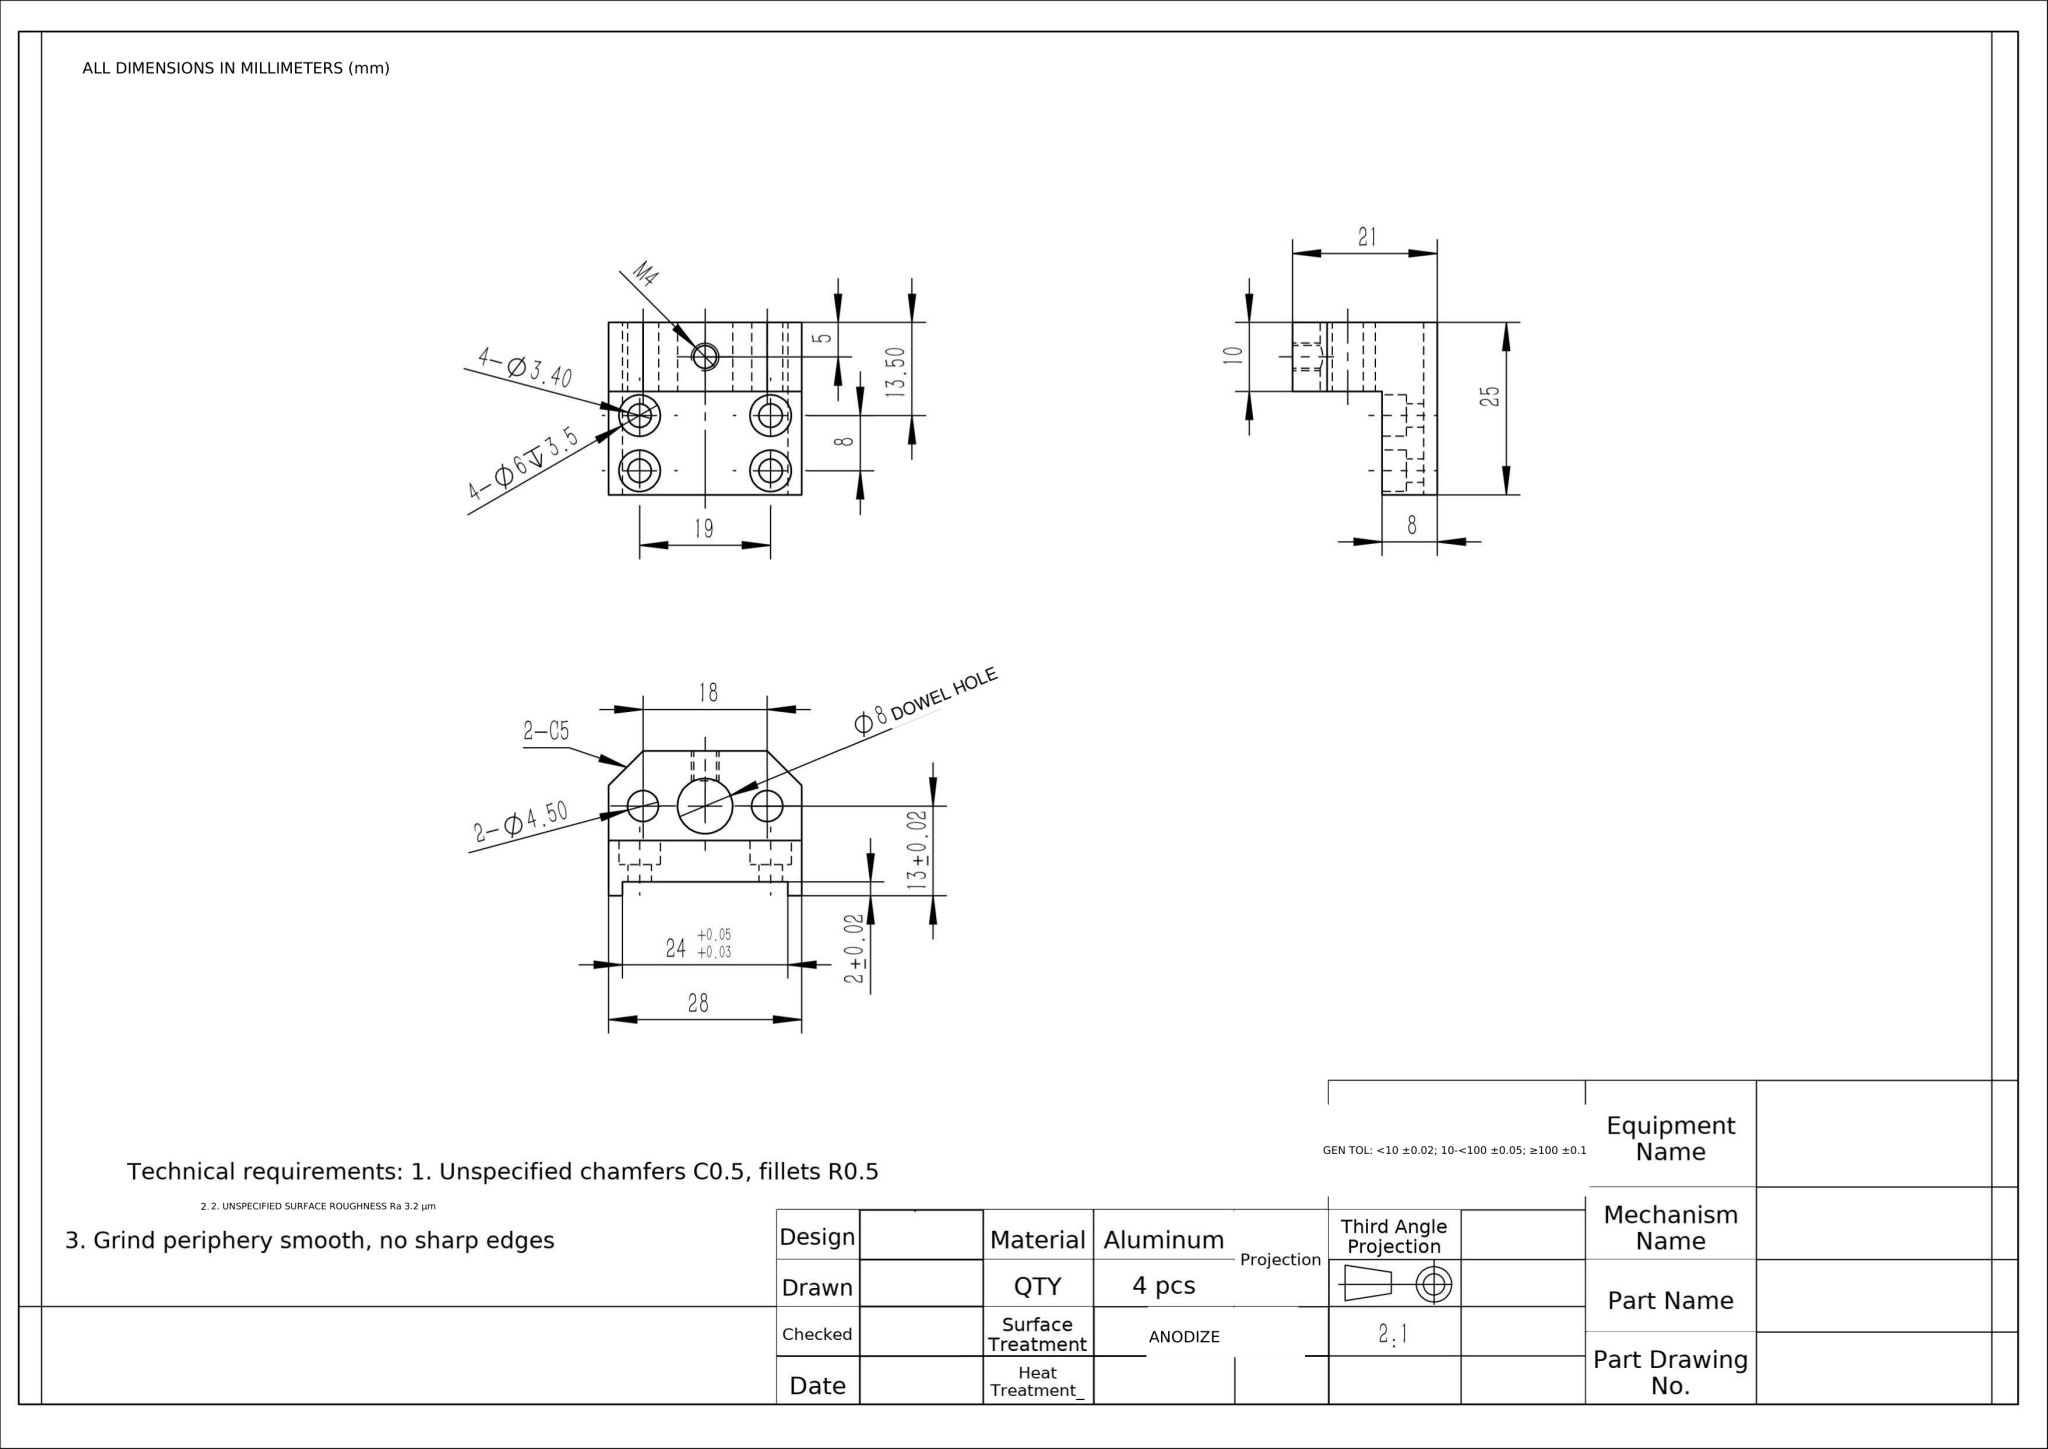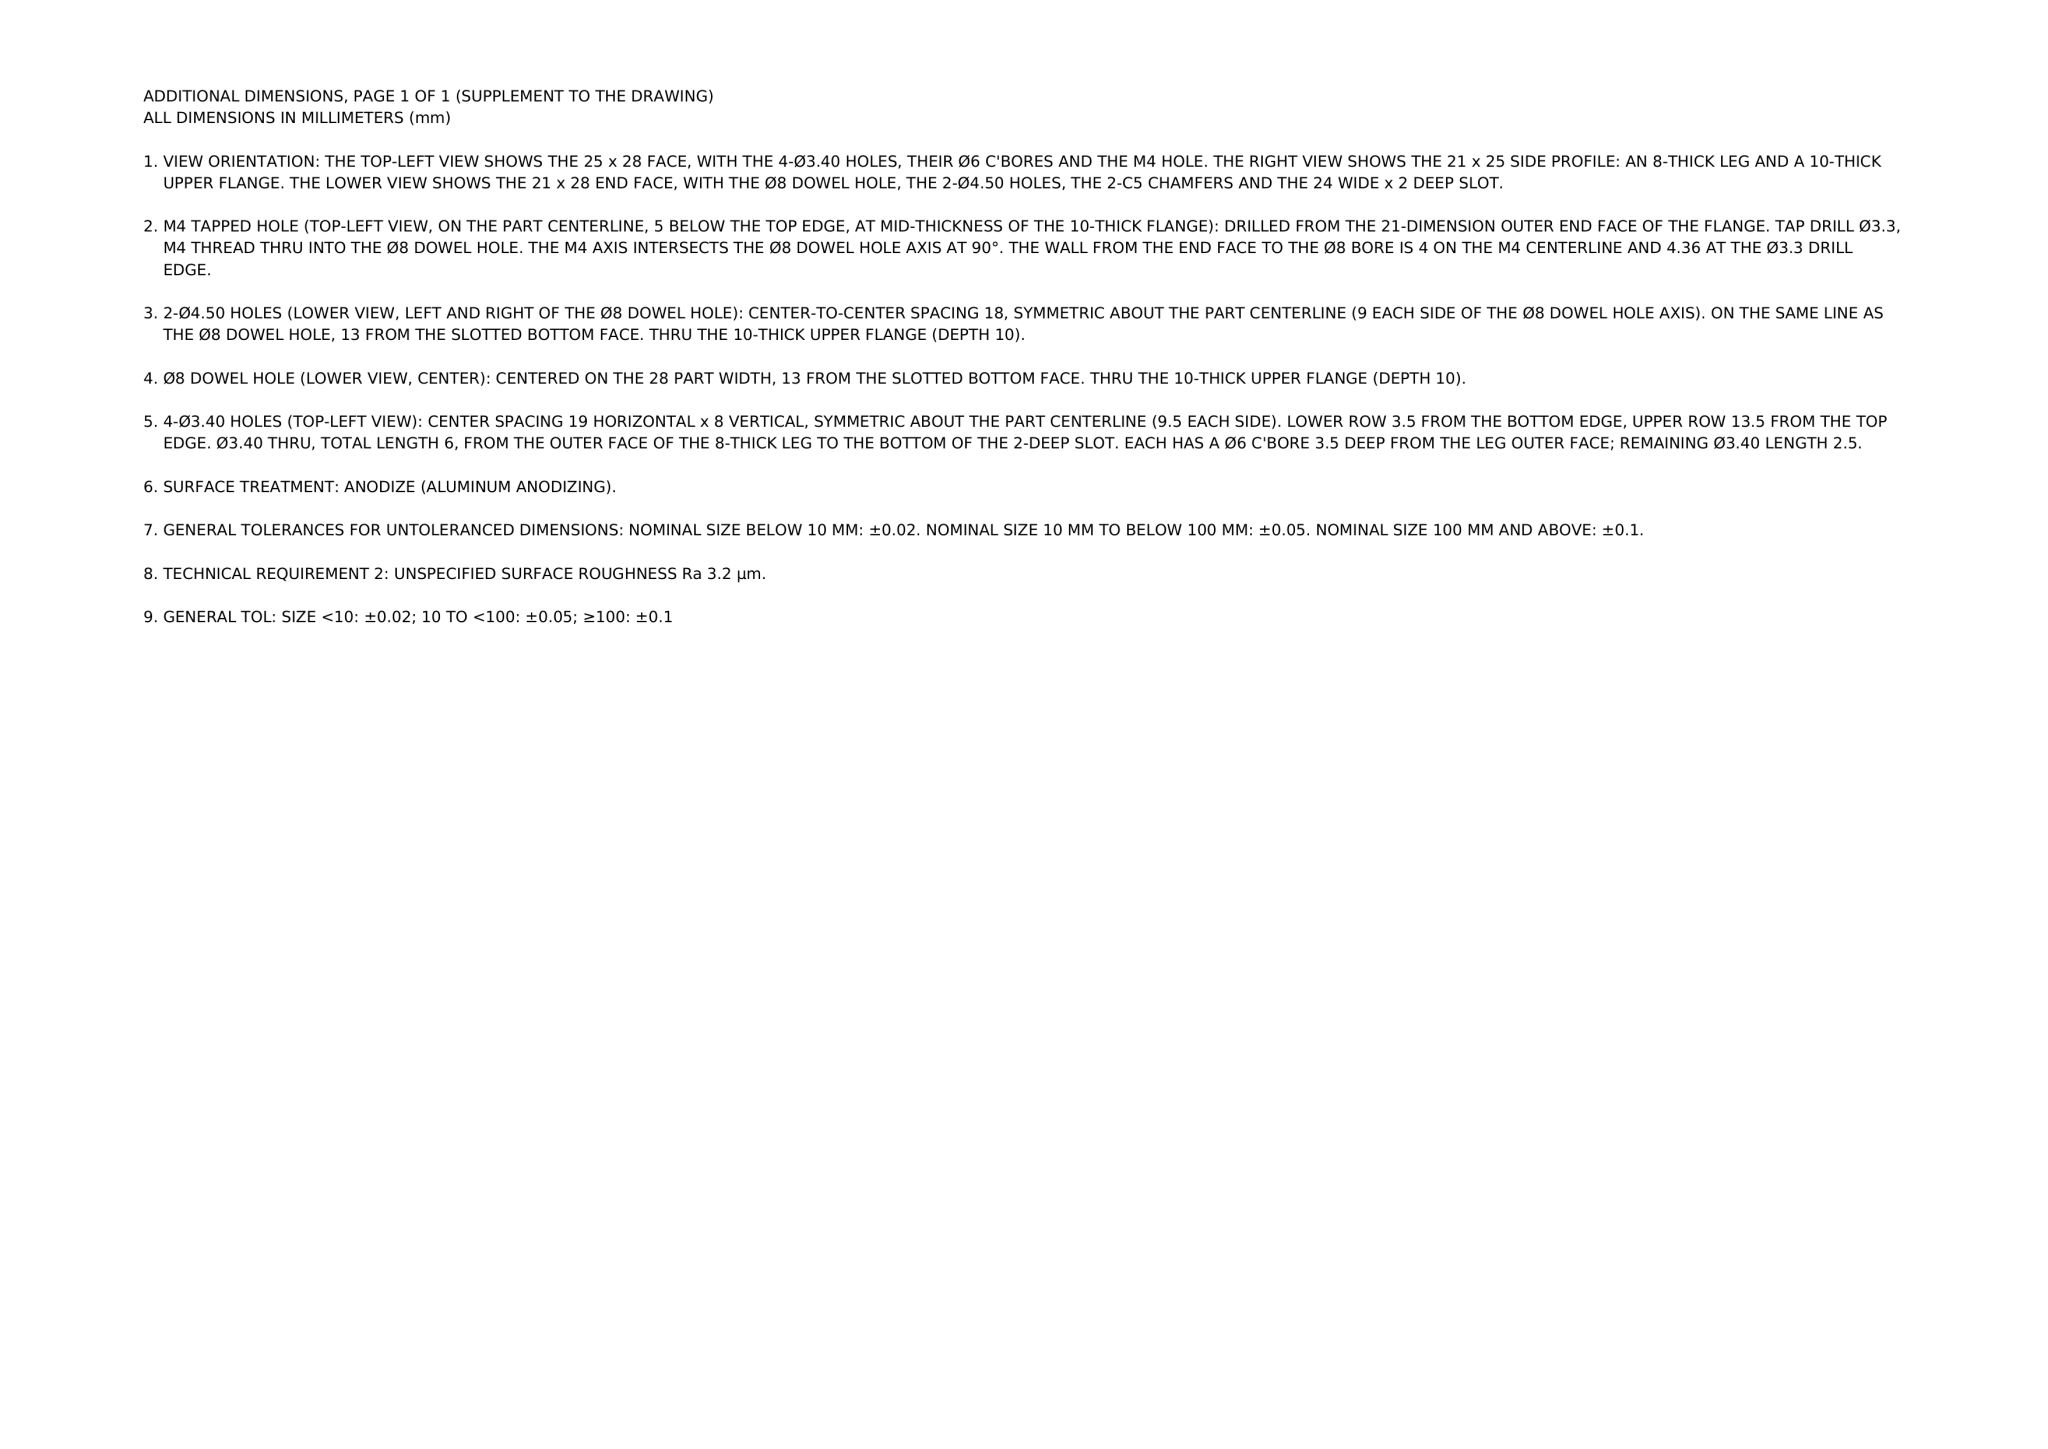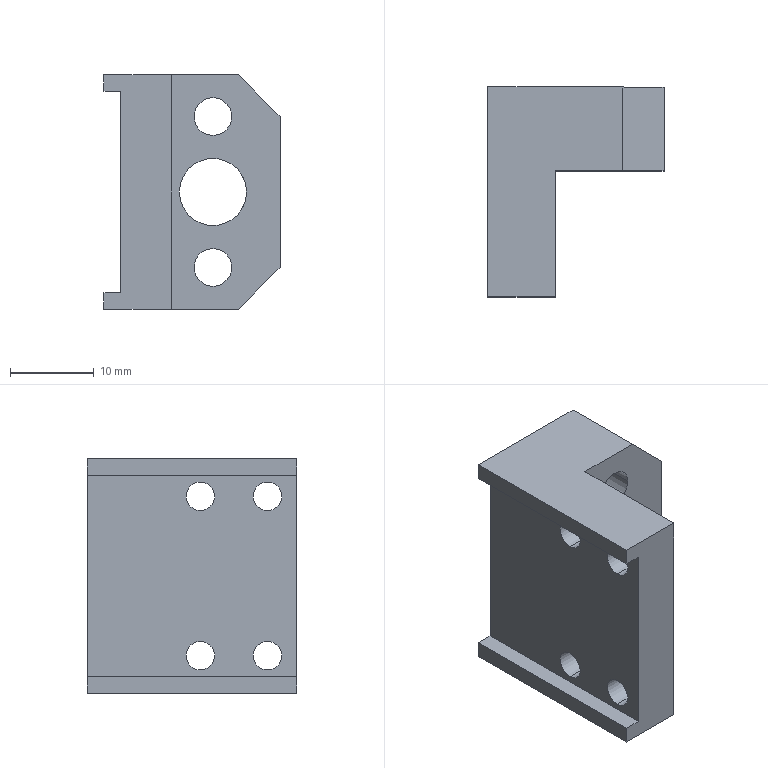Part | NX | mm | 1 solid | 42 faces | box 21 x 25 x 28 mm | volume 6448 mm3 | cylinder 24 | plane 18 | commonest cylinder face diameters 6 x8 3.4 x8 4.5 x4 3.3 x2 8 x2